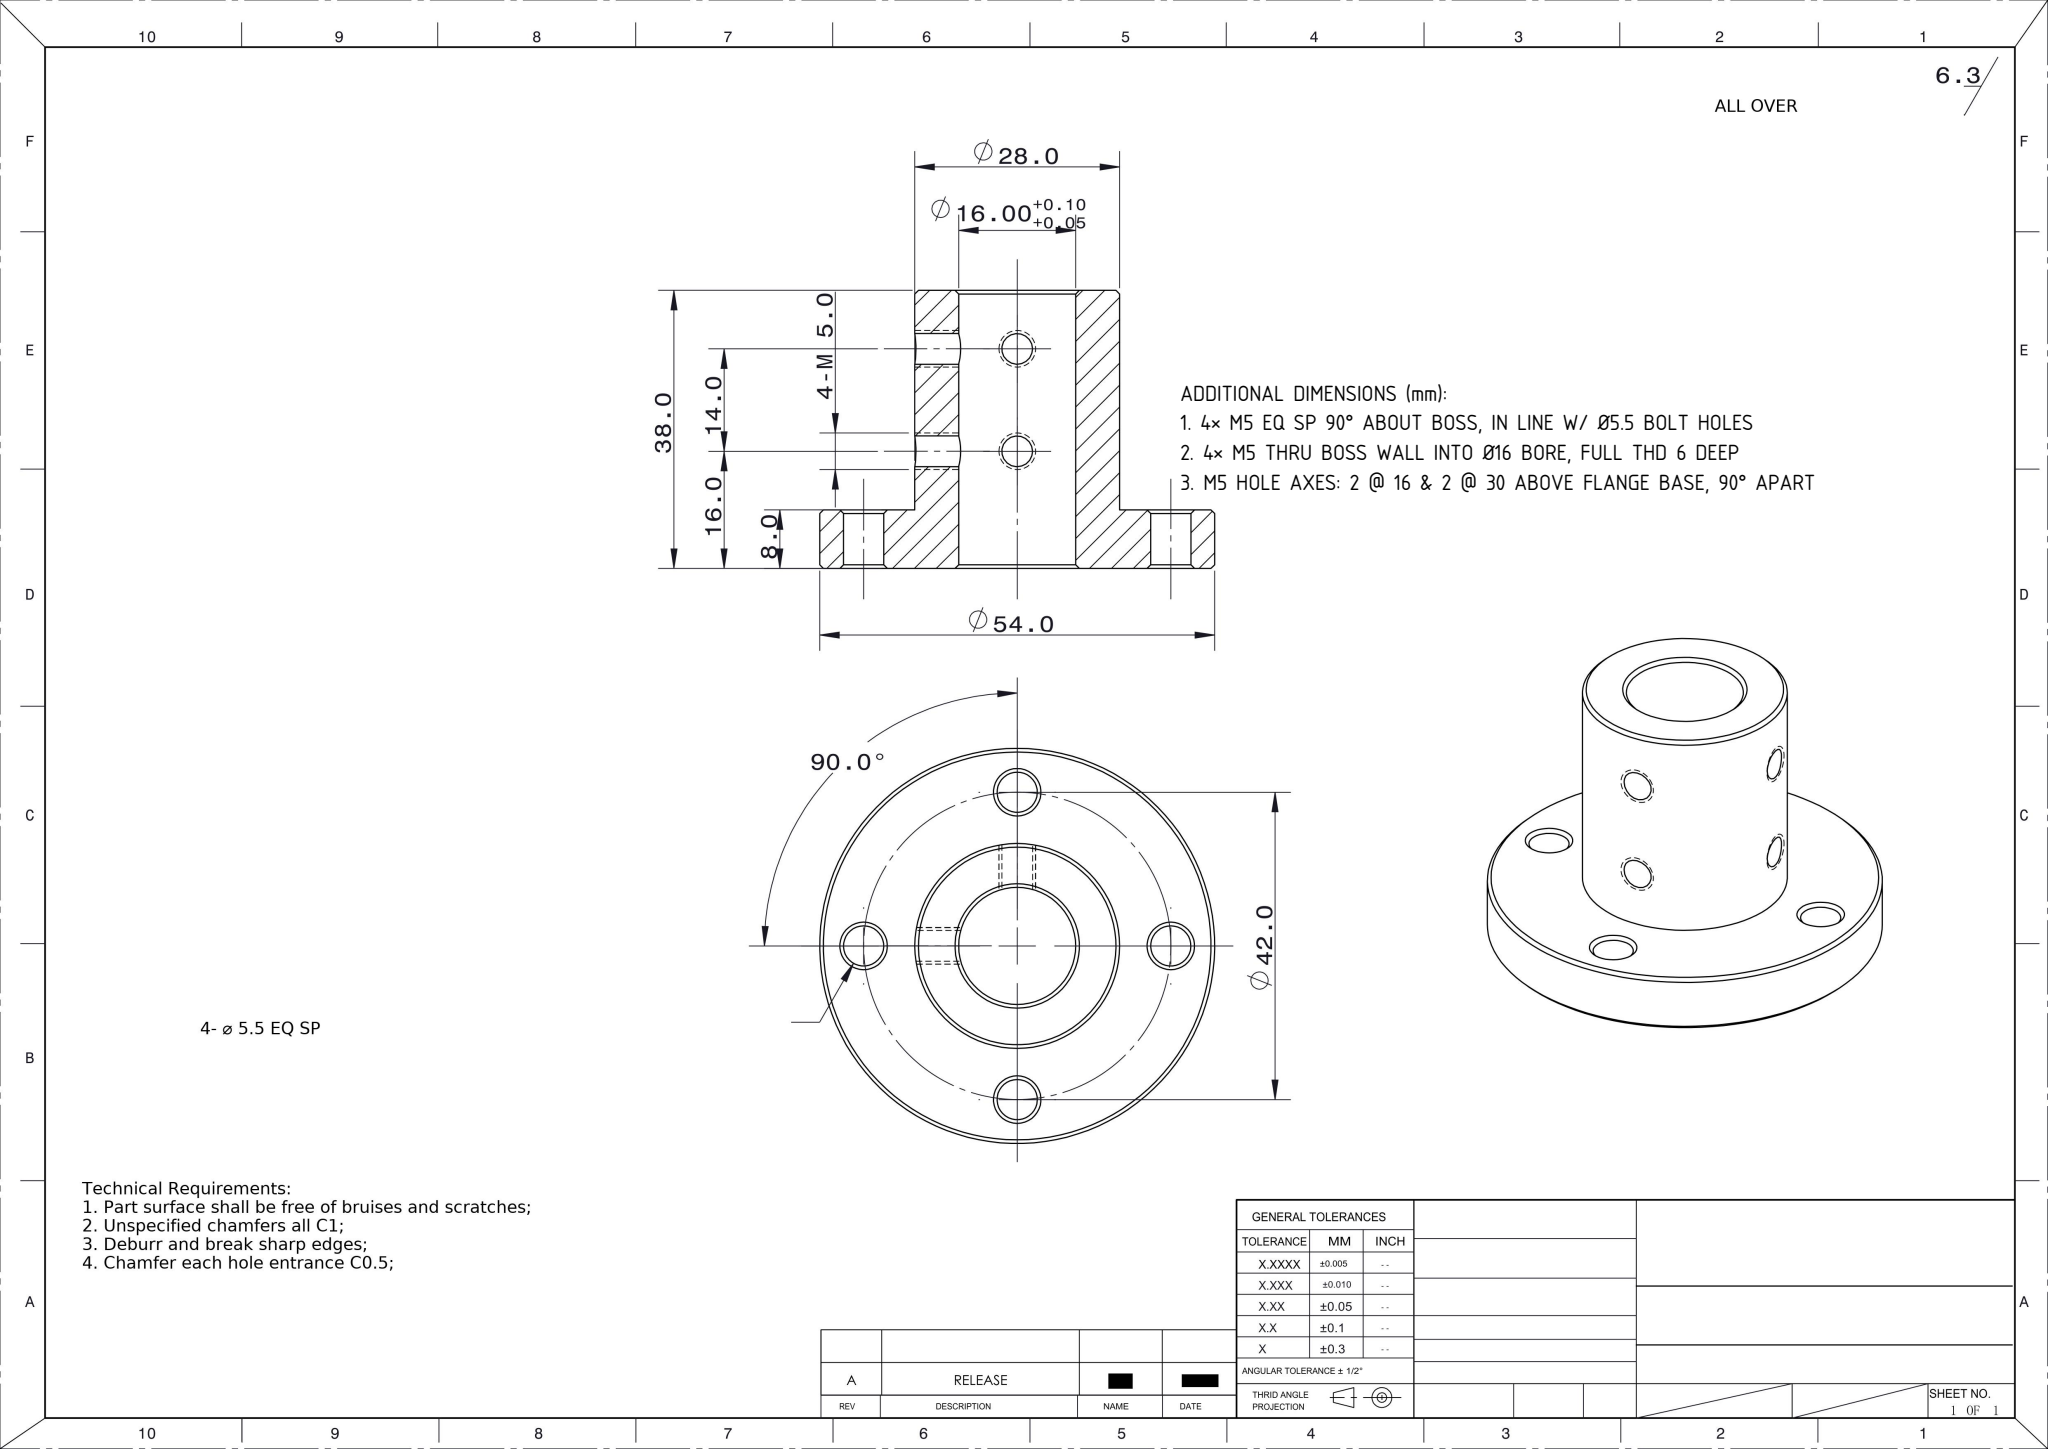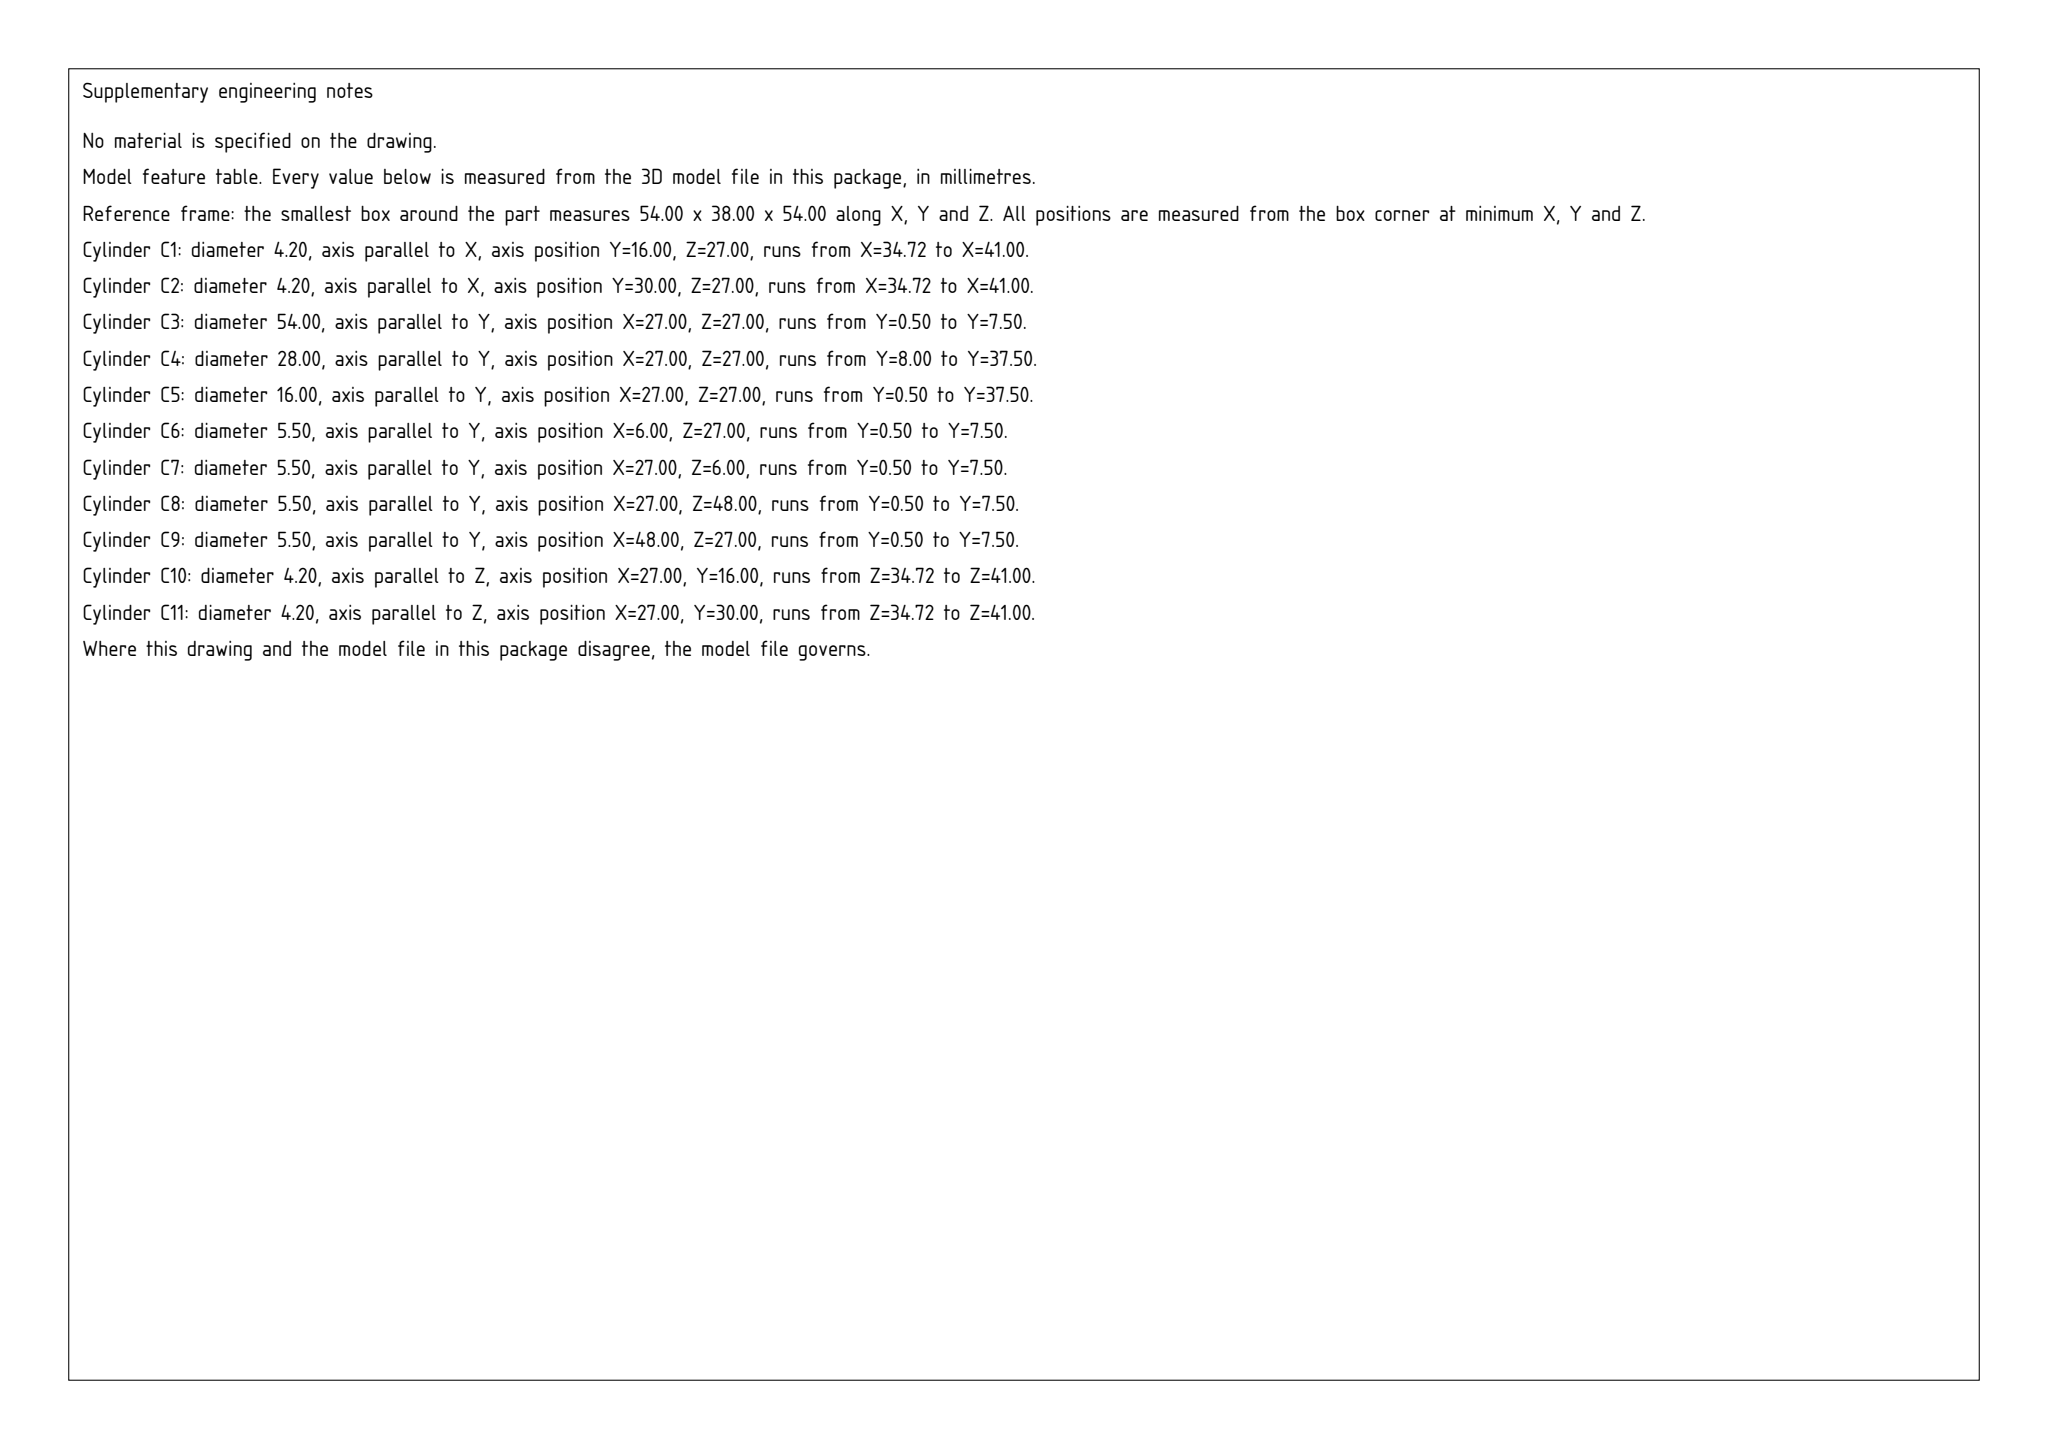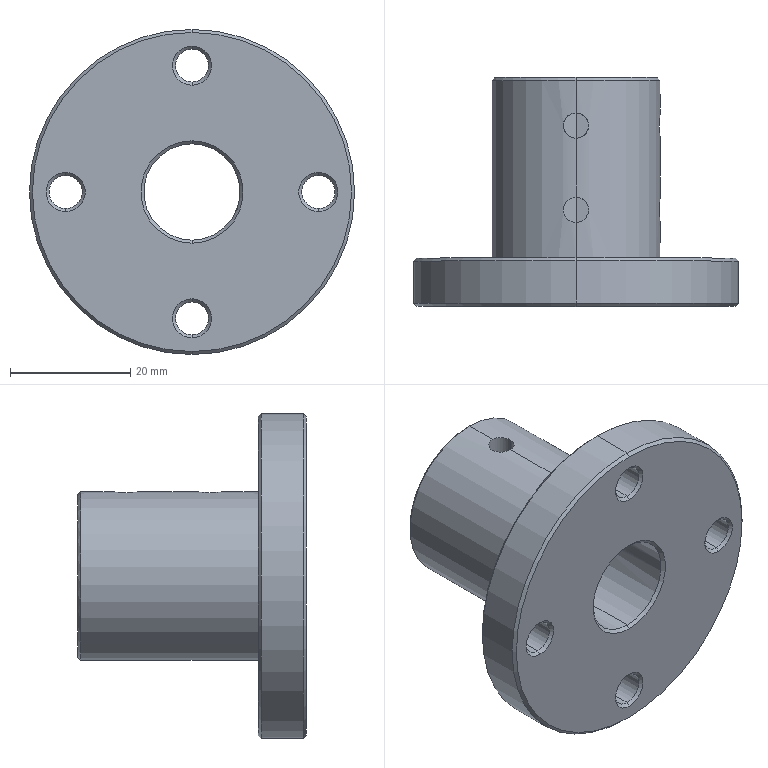Part | SolidWorks | mm | 1 solid | 51 faces | box 54 x 38 x 54 mm | volume 27975 mm3 | cone 26 | cylinder 22 | plane 3 | commonest cylinder face diameters 4.2 x8 5.5 x8 28 x2 54 x2 16 x2
build123d program:
from build123d import *

# Parameters (mm, degrees)
M5_CLEARANCE_HOLE1_D        = 5.5
SKETCH5_W                   = 2.1
SKETCH5_H                   = 27
M5_TAPPED_HOLE1_AT_2_COUNT  = 2
M5_TAPPED_HOLE1_AT_2_PITCH  = 14
CIRPATTERN1_COUNT           = 2
CIRPATTERN1_ANGLE           = 90
CIRPATTERN1_COPY_1_SKETCH_W = 2.1
CIRPATTERN1_COPY_1_SKETCH_H = 27
CHAMFER1_SIZE               = 0.5


with BuildPart() as part:
    # Sketch2 → Revolve1 (revolve)
    with BuildSketch(Plane.XY, mode=Mode.PRIVATE) as revolve1_sk:
        Polygon((8, 0), (8, -38), (27, -38), (27, -30), (14, -30), (14, 0), align=None)
    revolve(revolve1_sk.sketch.rotate(Axis((0, 0, 0), (0, 1, 0)), 90), axis=Axis((0, 0, 0), (0, 1, 0)))

    # M5 Clearance Hole1 (through all)
    with Locations(Plane(origin=(0, -30, 0), x_dir=(1, 0, 0), z_dir=(0, 1, 0))):
        with Locations((-21, 0), (0, 21), (0, -21), (21, 0)):
            Hole(M5_CLEARANCE_HOLE1_D / 2)

    # Sketch5 → M5 Tapped Hole1 (revolve, cut)
    with BuildSketch(Plane.ZX.offset(-8)):
        with Locations((1.05, 13.5)):
            Rectangle(SKETCH5_W, SKETCH5_H)
    m5_tapped_hole1 = revolve(axis=Axis((-6.35, -8, 0), (1, 0, 0)), mode=Mode.SUBTRACT)

    # M5 Tapped Hole1 at 2: M5 Tapped Hole1 ×2
    with Locations(*[(0, -i * M5_TAPPED_HOLE1_AT_2_PITCH, 0) for i in range(1, M5_TAPPED_HOLE1_AT_2_COUNT)]):
        add(m5_tapped_hole1, mode=Mode.SUBTRACT)

    # CirPattern1: M5 Tapped Hole1 ×2 about axis
    cirpattern1_axis = Axis((0, 0, 0), (0, -1, 0))
    for i in range(1, CIRPATTERN1_COUNT):
        add(m5_tapped_hole1.rotate(cirpattern1_axis, i * CIRPATTERN1_ANGLE / (CIRPATTERN1_COUNT - 1)), mode=Mode.SUBTRACT)

    # CirPattern1 copy 1 sketch → CirPattern1 copy 1 (revolve, cut)
    with BuildSketch(Plane(origin=(0, -22, 0), x_dir=(-1, 0, 0), z_dir=(0, 1, 0))):
        with Locations((1.05, 13.5)):
            Rectangle(CIRPATTERN1_COPY_1_SKETCH_W, CIRPATTERN1_COPY_1_SKETCH_H)
    revolve(axis=Axis((0, -22, -6.35), (0, 0, 1)), mode=Mode.SUBTRACT)

    # Chamfer1
    chamfer1_edges = [part.edges().sort_by_distance(p)[0] for p in [
        (23.75, -30, 0),
        (23.75, -38, 0),
        (2.75, -30, 21),
        (2.75, -38, 21),
        (2.75, -30, -21),
        (2.75, -38, -21),
        (-18.25, -30, 0),
        (-18.25, -38, 0),
        (0, 0, 14),
        (0, -30, 27),
        (0, -38, 27),
        (0, -38, 8),
        (0, 0, 8),
    ]]
    chamfer(chamfer1_edges, length=CHAMFER1_SIZE)


solid = part.part